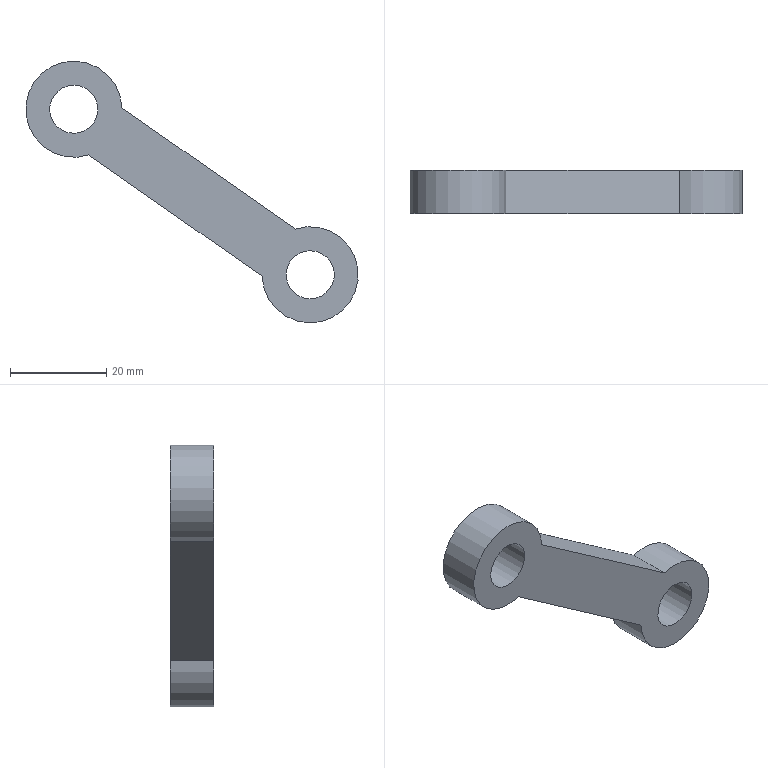Component | NX | CONNECTING_ROD_2 | 1 solid | 8 faces | box 69.15 x 9 x 54.41 mm | volume 8699 mm3 | cylinder 4 | plane 4 | commonest cylinder face diameters 20 x2 10 x2
STEP:
#1=CARTESIAN_POINT('',(0.,0.,0.));
#2=DIRECTION('',(0.,0.,1.));
#3=DIRECTION('',(1.,0.,0.));
#4=AXIS2_PLACEMENT_3D('',#1,#2,#3);
#5=CARTESIAN_POINT('',(-83.981,-59.005,124.741));
#6=VERTEX_POINT('',#5);
#7=CARTESIAN_POINT('',(-90.864,-59.005,114.911));
#8=VERTEX_POINT('',#7);
#9=CARTESIAN_POINT('',(-93.976,-59.005,124.415));
#10=DIRECTION('',(0.,-1.,0.));
#11=DIRECTION('',(0.8192,0.,-0.5736));
#12=AXIS2_PLACEMENT_3D('',#9,#10,#11);
#13=CIRCLE('',#12,10.);
#14=CARTESIAN_POINT('',(-93.976,-68.005,124.415));
#15=DIRECTION('',(0.,1.,0.));
#16=DIRECTION('',(-0.8192,0.,0.5736));
#17=AXIS2_PLACEMENT_3D('',#14,#15,#16);
#18=CYLINDRICAL_SURFACE('',#17,10.);
#19=CARTESIAN_POINT('',(3.142,9.));
#20=DIRECTION('',(-1.,0.));
#21=VECTOR('',#20,1.);
#22=LINE('',#19,#21);
#23=(GEOMETRIC_REPRESENTATION_CONTEXT(2)PARAMETRIC_REPRESENTATION_CONTEXT()REPRESENTATION_CONTEXT('',''));
#24=DEFINITIONAL_REPRESENTATION('',(#22),#23);
#25=PCURVE('',#18,#24);
#26=CARTESIAN_POINT('',(-93.976,-59.005,124.415));
#27=DIRECTION('',(0.,-1.,0.));
#28=DIRECTION('',(0.8192,0.,-0.5736));
#29=AXIS2_PLACEMENT_3D('',#26,#27,#28);
#30=PLANE('',#29);
#31=CARTESIAN_POINT('',(0.,0.));
#32=DIRECTION('',(1.,0.));
#33=AXIS2_PLACEMENT_2D('',#31,#32);
#34=CIRCLE('',#33,10.);
#35=(GEOMETRIC_REPRESENTATION_CONTEXT(2)PARAMETRIC_REPRESENTATION_CONTEXT()REPRESENTATION_CONTEXT('',''));
#36=DEFINITIONAL_REPRESENTATION('',(#34),#35);
#37=PCURVE('',#30,#36);
#38=SURFACE_CURVE('',#13,(#25,#37),.PCURVE_S1.);
#39=EDGE_CURVE('',#6,#8,#38,.T.);
#40=ORIENTED_EDGE('',*,*,#39,.T.);
#41=CARTESIAN_POINT('',(-90.864,-68.005,114.911));
#42=VERTEX_POINT('',#41);
#43=CARTESIAN_POINT('',(-90.864,-68.005,114.911));
#44=DIRECTION('',(0.,1.,0.));
#45=VECTOR('',#44,1.);
#46=LINE('',#43,#45);
#47=CARTESIAN_POINT('',(-2.498,0.));
#48=DIRECTION('',(0.,1.));
#49=VECTOR('',#48,1.);
#50=LINE('',#47,#49);
#51=(GEOMETRIC_REPRESENTATION_CONTEXT(2)PARAMETRIC_REPRESENTATION_CONTEXT()REPRESENTATION_CONTEXT('',''));
#52=DEFINITIONAL_REPRESENTATION('',(#50),#51);
#53=PCURVE('',#18,#52);
#54=CARTESIAN_POINT('',(-90.864,-68.005,114.911));
#55=DIRECTION('',(0.5736,0.,0.8192));
#56=DIRECTION('',(-0.8192,0.,0.5736));
#57=AXIS2_PLACEMENT_3D('',#54,#55,#56);
#58=PLANE('',#57);
#59=CARTESIAN_POINT('',(-0.,0.));
#60=DIRECTION('',(0.,-1.));
#61=VECTOR('',#60,1.);
#62=LINE('',#59,#61);
#63=(GEOMETRIC_REPRESENTATION_CONTEXT(2)PARAMETRIC_REPRESENTATION_CONTEXT()REPRESENTATION_CONTEXT('',''));
#64=DEFINITIONAL_REPRESENTATION('',(#62),#63);
#65=PCURVE('',#58,#64);
#66=SURFACE_CURVE('',#46,(#53,#65),.PCURVE_S1.);
#67=EDGE_CURVE('',#42,#8,#66,.T.);
#68=ORIENTED_EDGE('',*,*,#67,.F.);
#69=CARTESIAN_POINT('',(-83.981,-68.005,124.741));
#70=VERTEX_POINT('',#69);
#71=CARTESIAN_POINT('',(-93.976,-68.005,124.415));
#72=DIRECTION('',(0.,-1.,0.));
#73=DIRECTION('',(0.8192,0.,-0.5736));
#74=AXIS2_PLACEMENT_3D('',#71,#72,#73);
#75=CIRCLE('',#74,10.);
#76=CARTESIAN_POINT('',(3.142,0.));
#77=DIRECTION('',(-1.,0.));
#78=VECTOR('',#77,1.);
#79=LINE('',#76,#78);
#80=(GEOMETRIC_REPRESENTATION_CONTEXT(2)PARAMETRIC_REPRESENTATION_CONTEXT()REPRESENTATION_CONTEXT('',''));
#81=DEFINITIONAL_REPRESENTATION('',(#79),#80);
#82=PCURVE('',#18,#81);
#83=CARTESIAN_POINT('',(-93.976,-68.005,124.415));
#84=DIRECTION('',(0.,-1.,0.));
#85=DIRECTION('',(0.8192,0.,-0.5736));
#86=AXIS2_PLACEMENT_3D('',#83,#84,#85);
#87=PLANE('',#86);
#88=CARTESIAN_POINT('',(0.,0.));
#89=DIRECTION('',(1.,0.));
#90=AXIS2_PLACEMENT_2D('',#88,#89);
#91=CIRCLE('',#90,10.);
#92=(GEOMETRIC_REPRESENTATION_CONTEXT(2)PARAMETRIC_REPRESENTATION_CONTEXT()REPRESENTATION_CONTEXT('',''));
#93=DEFINITIONAL_REPRESENTATION('',(#91),#92);
#94=PCURVE('',#87,#93);
#95=SURFACE_CURVE('',#75,(#82,#94),.PCURVE_S1.);
#96=EDGE_CURVE('',#70,#42,#95,.T.);
#97=ORIENTED_EDGE('',*,*,#96,.F.);
#98=CARTESIAN_POINT('',(-83.981,-68.005,124.741));
#99=DIRECTION('',(0.,1.,0.));
#100=VECTOR('',#99,1.);
#101=LINE('',#98,#100);
#102=CARTESIAN_POINT('',(2.498,0.));
#103=DIRECTION('',(0.,1.));
#104=VECTOR('',#103,1.);
#105=LINE('',#102,#104);
#106=(GEOMETRIC_REPRESENTATION_CONTEXT(2)PARAMETRIC_REPRESENTATION_CONTEXT()REPRESENTATION_CONTEXT('',''));
#107=DEFINITIONAL_REPRESENTATION('',(#105),#106);
#108=PCURVE('',#18,#107);
#109=CARTESIAN_POINT('',(-47.938,-68.005,99.504));
#110=DIRECTION('',(-0.5736,0.,-0.8192));
#111=DIRECTION('',(0.8192,0.,-0.5736));
#112=AXIS2_PLACEMENT_3D('',#109,#110,#111);
#113=PLANE('',#112);
#114=CARTESIAN_POINT('',(-44.,0.));
#115=DIRECTION('',(0.,-1.));
#116=VECTOR('',#115,1.);
#117=LINE('',#114,#116);
#118=(GEOMETRIC_REPRESENTATION_CONTEXT(2)PARAMETRIC_REPRESENTATION_CONTEXT()REPRESENTATION_CONTEXT('',''));
#119=DEFINITIONAL_REPRESENTATION('',(#117),#118);
#120=PCURVE('',#113,#119);
#121=SURFACE_CURVE('',#101,(#108,#120),.PCURVE_S1.);
#122=EDGE_CURVE('',#70,#6,#121,.T.);
#123=ORIENTED_EDGE('',*,*,#122,.T.);
#124=EDGE_LOOP('',(#40,#68,#97,#123));
#125=FACE_BOUND('',#124,.T.);
#126=ADVANCED_FACE('',(#125),#18,.T.);
#127=CARTESIAN_POINT('',(-54.821,-59.005,89.674));
#128=VERTEX_POINT('',#127);
#129=CARTESIAN_POINT('',(-90.864,-59.005,114.911));
#130=DIRECTION('',(0.8192,0.,-0.5736));
#131=VECTOR('',#130,1.);
#132=LINE('',#129,#131);
#133=CARTESIAN_POINT('',(0.,-9.));
#134=DIRECTION('',(-1.,0.));
#135=VECTOR('',#134,1.);
#136=LINE('',#133,#135);
#137=(GEOMETRIC_REPRESENTATION_CONTEXT(2)PARAMETRIC_REPRESENTATION_CONTEXT()REPRESENTATION_CONTEXT('',''));
#138=DEFINITIONAL_REPRESENTATION('',(#136),#137);
#139=PCURVE('',#58,#138);
#140=CARTESIAN_POINT('',(8.,-6.));
#141=DIRECTION('',(1.,0.));
#142=VECTOR('',#141,1.);
#143=LINE('',#140,#142);
#144=(GEOMETRIC_REPRESENTATION_CONTEXT(2)PARAMETRIC_REPRESENTATION_CONTEXT()REPRESENTATION_CONTEXT('',''));
#145=DEFINITIONAL_REPRESENTATION('',(#143),#144);
#146=PCURVE('',#30,#145);
#147=SURFACE_CURVE('',#132,(#139,#146),.PCURVE_S1.);
#148=EDGE_CURVE('',#8,#128,#147,.T.);
#149=ORIENTED_EDGE('',*,*,#148,.T.);
#150=CARTESIAN_POINT('',(-54.821,-68.005,89.674));
#151=VERTEX_POINT('',#150);
#152=CARTESIAN_POINT('',(-54.821,-68.005,89.674));
#153=DIRECTION('',(0.,1.,0.));
#154=VECTOR('',#153,1.);
#155=LINE('',#152,#154);
#156=CARTESIAN_POINT('',(-44.,0.));
#157=DIRECTION('',(0.,-1.));
#158=VECTOR('',#157,1.);
#159=LINE('',#156,#158);
#160=(GEOMETRIC_REPRESENTATION_CONTEXT(2)PARAMETRIC_REPRESENTATION_CONTEXT()REPRESENTATION_CONTEXT('',''));
#161=DEFINITIONAL_REPRESENTATION('',(#159),#160);
#162=PCURVE('',#58,#161);
#163=CARTESIAN_POINT('',(-44.827,-68.005,90.));
#164=DIRECTION('',(0.,1.,0.));
#165=DIRECTION('',(-0.8192,0.,0.5736));
#166=AXIS2_PLACEMENT_3D('',#163,#164,#165);
#167=CYLINDRICAL_SURFACE('',#166,10.);
#168=CARTESIAN_POINT('',(5.64,0.));
#169=DIRECTION('',(0.,1.));
#170=VECTOR('',#169,1.);
#171=LINE('',#168,#170);
#172=(GEOMETRIC_REPRESENTATION_CONTEXT(2)PARAMETRIC_REPRESENTATION_CONTEXT()REPRESENTATION_CONTEXT('',''));
#173=DEFINITIONAL_REPRESENTATION('',(#171),#172);
#174=PCURVE('',#167,#173);
#175=SURFACE_CURVE('',#155,(#162,#174),.PCURVE_S1.);
#176=EDGE_CURVE('',#151,#128,#175,.T.);
#177=ORIENTED_EDGE('',*,*,#176,.F.);
#178=CARTESIAN_POINT('',(-90.864,-68.005,114.911));
#179=DIRECTION('',(0.8192,0.,-0.5736));
#180=VECTOR('',#179,1.);
#181=LINE('',#178,#180);
#182=CARTESIAN_POINT('',(0.,0.));
#183=DIRECTION('',(-1.,0.));
#184=VECTOR('',#183,1.);
#185=LINE('',#182,#184);
#186=(GEOMETRIC_REPRESENTATION_CONTEXT(2)PARAMETRIC_REPRESENTATION_CONTEXT()REPRESENTATION_CONTEXT('',''));
#187=DEFINITIONAL_REPRESENTATION('',(#185),#186);
#188=PCURVE('',#58,#187);
#189=CARTESIAN_POINT('',(8.,-6.));
#190=DIRECTION('',(1.,0.));
#191=VECTOR('',#190,1.);
#192=LINE('',#189,#191);
#193=(GEOMETRIC_REPRESENTATION_CONTEXT(2)PARAMETRIC_REPRESENTATION_CONTEXT()REPRESENTATION_CONTEXT('',''));
#194=DEFINITIONAL_REPRESENTATION('',(#192),#193);
#195=PCURVE('',#87,#194);
#196=SURFACE_CURVE('',#181,(#188,#195),.PCURVE_S1.);
#197=EDGE_CURVE('',#42,#151,#196,.T.);
#198=ORIENTED_EDGE('',*,*,#197,.F.);
#199=ORIENTED_EDGE('',*,*,#67,.T.);
#200=EDGE_LOOP('',(#149,#177,#198,#199));
#201=FACE_BOUND('',#200,.T.);
#202=ADVANCED_FACE('',(#201),#58,.F.);
#203=CARTESIAN_POINT('',(-47.938,-59.005,99.504));
#204=VERTEX_POINT('',#203);
#205=CARTESIAN_POINT('',(-44.827,-59.005,90.));
#206=DIRECTION('',(0.,-1.,0.));
#207=DIRECTION('',(0.8192,0.,-0.5736));
#208=AXIS2_PLACEMENT_3D('',#205,#206,#207);
#209=CIRCLE('',#208,10.);
#210=CARTESIAN_POINT('',(9.425,9.));
#211=DIRECTION('',(-1.,0.));
#212=VECTOR('',#211,1.);
#213=LINE('',#210,#212);
#214=(GEOMETRIC_REPRESENTATION_CONTEXT(2)PARAMETRIC_REPRESENTATION_CONTEXT()REPRESENTATION_CONTEXT('',''));
#215=DEFINITIONAL_REPRESENTATION('',(#213),#214);
#216=PCURVE('',#167,#215);
#217=CARTESIAN_POINT('',(60.,-0.));
#218=DIRECTION('',(1.,0.));
#219=AXIS2_PLACEMENT_2D('',#217,#218);
#220=CIRCLE('',#219,10.);
#221=(GEOMETRIC_REPRESENTATION_CONTEXT(2)PARAMETRIC_REPRESENTATION_CONTEXT()REPRESENTATION_CONTEXT('',''));
#222=DEFINITIONAL_REPRESENTATION('',(#220),#221);
#223=PCURVE('',#30,#222);
#224=SURFACE_CURVE('',#209,(#216,#223),.PCURVE_S1.);
#225=EDGE_CURVE('',#128,#204,#224,.T.);
#226=ORIENTED_EDGE('',*,*,#225,.T.);
#227=CARTESIAN_POINT('',(-47.938,-68.005,99.504));
#228=VERTEX_POINT('',#227);
#229=CARTESIAN_POINT('',(-47.938,-68.005,99.504));
#230=DIRECTION('',(0.,1.,0.));
#231=VECTOR('',#230,1.);
#232=LINE('',#229,#231);
#233=CARTESIAN_POINT('',(0.6435,0.));
#234=DIRECTION('',(0.,1.));
#235=VECTOR('',#234,1.);
#236=LINE('',#233,#235);
#237=(GEOMETRIC_REPRESENTATION_CONTEXT(2)PARAMETRIC_REPRESENTATION_CONTEXT()REPRESENTATION_CONTEXT('',''));
#238=DEFINITIONAL_REPRESENTATION('',(#236),#237);
#239=PCURVE('',#167,#238);
#240=CARTESIAN_POINT('',(0.,0.));
#241=DIRECTION('',(0.,-1.));
#242=VECTOR('',#241,1.);
#243=LINE('',#240,#242);
#244=(GEOMETRIC_REPRESENTATION_CONTEXT(2)PARAMETRIC_REPRESENTATION_CONTEXT()REPRESENTATION_CONTEXT('',''));
#245=DEFINITIONAL_REPRESENTATION('',(#243),#244);
#246=PCURVE('',#113,#245);
#247=SURFACE_CURVE('',#232,(#239,#246),.PCURVE_S1.);
#248=EDGE_CURVE('',#228,#204,#247,.T.);
#249=ORIENTED_EDGE('',*,*,#248,.F.);
#250=CARTESIAN_POINT('',(-44.827,-68.005,90.));
#251=DIRECTION('',(0.,-1.,0.));
#252=DIRECTION('',(0.8192,0.,-0.5736));
#253=AXIS2_PLACEMENT_3D('',#250,#251,#252);
#254=CIRCLE('',#253,10.);
#255=CARTESIAN_POINT('',(9.425,0.));
#256=DIRECTION('',(-1.,0.));
#257=VECTOR('',#256,1.);
#258=LINE('',#255,#257);
#259=(GEOMETRIC_REPRESENTATION_CONTEXT(2)PARAMETRIC_REPRESENTATION_CONTEXT()REPRESENTATION_CONTEXT('',''));
#260=DEFINITIONAL_REPRESENTATION('',(#258),#259);
#261=PCURVE('',#167,#260);
#262=CARTESIAN_POINT('',(60.,-0.));
#263=DIRECTION('',(1.,0.));
#264=AXIS2_PLACEMENT_2D('',#262,#263);
#265=CIRCLE('',#264,10.);
#266=(GEOMETRIC_REPRESENTATION_CONTEXT(2)PARAMETRIC_REPRESENTATION_CONTEXT()REPRESENTATION_CONTEXT('',''));
#267=DEFINITIONAL_REPRESENTATION('',(#265),#266);
#268=PCURVE('',#87,#267);
#269=SURFACE_CURVE('',#254,(#261,#268),.PCURVE_S1.);
#270=EDGE_CURVE('',#151,#228,#269,.T.);
#271=ORIENTED_EDGE('',*,*,#270,.F.);
#272=ORIENTED_EDGE('',*,*,#176,.T.);
#273=EDGE_LOOP('',(#226,#249,#271,#272));
#274=FACE_BOUND('',#273,.T.);
#275=ADVANCED_FACE('',(#274),#167,.T.);
#276=CARTESIAN_POINT('',(-89.88,-68.005,121.547));
#277=VERTEX_POINT('',#276);
#278=CARTESIAN_POINT('',(-93.976,-68.005,124.415));
#279=DIRECTION('',(0.,-1.,0.));
#280=DIRECTION('',(0.8192,0.,-0.5736));
#281=AXIS2_PLACEMENT_3D('',#278,#279,#280);
#282=CIRCLE('',#281,5.);
#283=CARTESIAN_POINT('',(-93.976,-68.005,124.415));
#284=DIRECTION('',(0.,1.,0.));
#285=DIRECTION('',(-0.8192,0.,0.5736));
#286=AXIS2_PLACEMENT_3D('',#283,#284,#285);
#287=CYLINDRICAL_SURFACE('',#286,5.);
#288=CARTESIAN_POINT('',(9.425,0.));
#289=DIRECTION('',(-1.,0.));
#290=VECTOR('',#289,1.);
#291=LINE('',#288,#290);
#292=(GEOMETRIC_REPRESENTATION_CONTEXT(2)PARAMETRIC_REPRESENTATION_CONTEXT()REPRESENTATION_CONTEXT('',''));
#293=DEFINITIONAL_REPRESENTATION('',(#291),#292);
#294=PCURVE('',#287,#293);
#295=CARTESIAN_POINT('',(0.,0.));
#296=DIRECTION('',(1.,0.));
#297=AXIS2_PLACEMENT_2D('',#295,#296);
#298=CIRCLE('',#297,5.);
#299=(GEOMETRIC_REPRESENTATION_CONTEXT(2)PARAMETRIC_REPRESENTATION_CONTEXT()REPRESENTATION_CONTEXT('',''));
#300=DEFINITIONAL_REPRESENTATION('',(#298),#299);
#301=PCURVE('',#87,#300);
#302=SURFACE_CURVE('',#282,(#294,#301),.PCURVE_S1.);
#303=EDGE_CURVE('',#277,#277,#302,.T.);
#304=ORIENTED_EDGE('',*,*,#303,.F.);
#305=CARTESIAN_POINT('',(-89.88,-59.005,121.547));
#306=VERTEX_POINT('',#305);
#307=CARTESIAN_POINT('',(-89.88,-68.005,121.547));
#308=CARTESIAN_POINT('',(-89.88,-59.005,121.547));
#309=B_SPLINE_CURVE_WITH_KNOTS('',1,(#307,#308),.UNSPECIFIED.,.F.,.F.,(2,2),(0.,9.),.PIECEWISE_BEZIER_KNOTS.);
#310=CARTESIAN_POINT('',(9.425,0.));
#311=DIRECTION('',(0.,1.));
#312=VECTOR('',#311,1.);
#313=LINE('',#310,#312);
#314=(GEOMETRIC_REPRESENTATION_CONTEXT(2)PARAMETRIC_REPRESENTATION_CONTEXT()REPRESENTATION_CONTEXT('',''));
#315=DEFINITIONAL_REPRESENTATION('',(#313),#314);
#316=PCURVE('',#287,#315);
#317=CARTESIAN_POINT('',(3.142,0.));
#318=DIRECTION('',(0.,1.));
#319=VECTOR('',#318,1.);
#320=LINE('',#317,#319);
#321=(GEOMETRIC_REPRESENTATION_CONTEXT(2)PARAMETRIC_REPRESENTATION_CONTEXT()REPRESENTATION_CONTEXT('',''));
#322=DEFINITIONAL_REPRESENTATION('',(#320),#321);
#323=PCURVE('',#287,#322);
#324=SEAM_CURVE('',#309,(#316,#323),.PCURVE_S1.);
#325=EDGE_CURVE('',#277,#306,#324,.T.);
#326=ORIENTED_EDGE('',*,*,#325,.T.);
#327=CARTESIAN_POINT('',(-93.976,-59.005,124.415));
#328=DIRECTION('',(0.,-1.,0.));
#329=DIRECTION('',(0.8192,0.,-0.5736));
#330=AXIS2_PLACEMENT_3D('',#327,#328,#329);
#331=CIRCLE('',#330,5.);
#332=CARTESIAN_POINT('',(9.425,9.));
#333=DIRECTION('',(-1.,0.));
#334=VECTOR('',#333,1.);
#335=LINE('',#332,#334);
#336=(GEOMETRIC_REPRESENTATION_CONTEXT(2)PARAMETRIC_REPRESENTATION_CONTEXT()REPRESENTATION_CONTEXT('',''));
#337=DEFINITIONAL_REPRESENTATION('',(#335),#336);
#338=PCURVE('',#287,#337);
#339=CARTESIAN_POINT('',(0.,0.));
#340=DIRECTION('',(1.,0.));
#341=AXIS2_PLACEMENT_2D('',#339,#340);
#342=CIRCLE('',#341,5.);
#343=(GEOMETRIC_REPRESENTATION_CONTEXT(2)PARAMETRIC_REPRESENTATION_CONTEXT()REPRESENTATION_CONTEXT('',''));
#344=DEFINITIONAL_REPRESENTATION('',(#342),#343);
#345=PCURVE('',#30,#344);
#346=SURFACE_CURVE('',#331,(#338,#345),.PCURVE_S1.);
#347=EDGE_CURVE('',#306,#306,#346,.T.);
#348=ORIENTED_EDGE('',*,*,#347,.T.);
#349=ORIENTED_EDGE('',*,*,#325,.F.);
#350=EDGE_LOOP('',(#304,#326,#348,#349));
#351=FACE_BOUND('',#350,.F.);
#352=ADVANCED_FACE('',(#351),#287,.F.);
#353=CARTESIAN_POINT('',(-47.938,-59.005,99.504));
#354=DIRECTION('',(-0.8192,0.,0.5736));
#355=VECTOR('',#354,1.);
#356=LINE('',#353,#355);
#357=CARTESIAN_POINT('',(0.,-9.));
#358=DIRECTION('',(-1.,0.));
#359=VECTOR('',#358,1.);
#360=LINE('',#357,#359);
#361=(GEOMETRIC_REPRESENTATION_CONTEXT(2)PARAMETRIC_REPRESENTATION_CONTEXT()REPRESENTATION_CONTEXT('',''));
#362=DEFINITIONAL_REPRESENTATION('',(#360),#361);
#363=PCURVE('',#113,#362);
#364=CARTESIAN_POINT('',(52.,6.));
#365=DIRECTION('',(-1.,0.));
#366=VECTOR('',#365,1.);
#367=LINE('',#364,#366);
#368=(GEOMETRIC_REPRESENTATION_CONTEXT(2)PARAMETRIC_REPRESENTATION_CONTEXT()REPRESENTATION_CONTEXT('',''));
#369=DEFINITIONAL_REPRESENTATION('',(#367),#368);
#370=PCURVE('',#30,#369);
#371=SURFACE_CURVE('',#356,(#363,#370),.PCURVE_S1.);
#372=EDGE_CURVE('',#204,#6,#371,.T.);
#373=ORIENTED_EDGE('',*,*,#372,.T.);
#374=ORIENTED_EDGE('',*,*,#122,.F.);
#375=CARTESIAN_POINT('',(-47.938,-68.005,99.504));
#376=DIRECTION('',(-0.8192,0.,0.5736));
#377=VECTOR('',#376,1.);
#378=LINE('',#375,#377);
#379=CARTESIAN_POINT('',(0.,0.));
#380=DIRECTION('',(-1.,0.));
#381=VECTOR('',#380,1.);
#382=LINE('',#379,#381);
#383=(GEOMETRIC_REPRESENTATION_CONTEXT(2)PARAMETRIC_REPRESENTATION_CONTEXT()REPRESENTATION_CONTEXT('',''));
#384=DEFINITIONAL_REPRESENTATION('',(#382),#383);
#385=PCURVE('',#113,#384);
#386=CARTESIAN_POINT('',(52.,6.));
#387=DIRECTION('',(-1.,0.));
#388=VECTOR('',#387,1.);
#389=LINE('',#386,#388);
#390=(GEOMETRIC_REPRESENTATION_CONTEXT(2)PARAMETRIC_REPRESENTATION_CONTEXT()REPRESENTATION_CONTEXT('',''));
#391=DEFINITIONAL_REPRESENTATION('',(#389),#390);
#392=PCURVE('',#87,#391);
#393=SURFACE_CURVE('',#378,(#385,#392),.PCURVE_S1.);
#394=EDGE_CURVE('',#228,#70,#393,.T.);
#395=ORIENTED_EDGE('',*,*,#394,.F.);
#396=ORIENTED_EDGE('',*,*,#248,.T.);
#397=EDGE_LOOP('',(#373,#374,#395,#396));
#398=FACE_BOUND('',#397,.T.);
#399=ADVANCED_FACE('',(#398),#113,.F.);
#400=CARTESIAN_POINT('',(-40.731,-68.005,87.132));
#401=VERTEX_POINT('',#400);
#402=CARTESIAN_POINT('',(-44.827,-68.005,90.));
#403=DIRECTION('',(0.,-1.,0.));
#404=DIRECTION('',(0.8192,0.,-0.5736));
#405=AXIS2_PLACEMENT_3D('',#402,#403,#404);
#406=CIRCLE('',#405,5.);
#407=CARTESIAN_POINT('',(-44.827,-68.005,90.));
#408=DIRECTION('',(0.,1.,0.));
#409=DIRECTION('',(-0.8192,0.,0.5736));
#410=AXIS2_PLACEMENT_3D('',#407,#408,#409);
#411=CYLINDRICAL_SURFACE('',#410,5.);
#412=CARTESIAN_POINT('',(9.425,0.));
#413=DIRECTION('',(-1.,0.));
#414=VECTOR('',#413,1.);
#415=LINE('',#412,#414);
#416=(GEOMETRIC_REPRESENTATION_CONTEXT(2)PARAMETRIC_REPRESENTATION_CONTEXT()REPRESENTATION_CONTEXT('',''));
#417=DEFINITIONAL_REPRESENTATION('',(#415),#416);
#418=PCURVE('',#411,#417);
#419=CARTESIAN_POINT('',(60.,-0.));
#420=DIRECTION('',(1.,0.));
#421=AXIS2_PLACEMENT_2D('',#419,#420);
#422=CIRCLE('',#421,5.);
#423=(GEOMETRIC_REPRESENTATION_CONTEXT(2)PARAMETRIC_REPRESENTATION_CONTEXT()REPRESENTATION_CONTEXT('',''));
#424=DEFINITIONAL_REPRESENTATION('',(#422),#423);
#425=PCURVE('',#87,#424);
#426=SURFACE_CURVE('',#406,(#418,#425),.PCURVE_S1.);
#427=EDGE_CURVE('',#401,#401,#426,.T.);
#428=ORIENTED_EDGE('',*,*,#427,.F.);
#429=CARTESIAN_POINT('',(-40.731,-59.005,87.132));
#430=VERTEX_POINT('',#429);
#431=CARTESIAN_POINT('',(-40.731,-68.005,87.132));
#432=CARTESIAN_POINT('',(-40.731,-59.005,87.132));
#433=B_SPLINE_CURVE_WITH_KNOTS('',1,(#431,#432),.UNSPECIFIED.,.F.,.F.,(2,2),(0.,9.),.PIECEWISE_BEZIER_KNOTS.);
#434=CARTESIAN_POINT('',(9.425,0.));
#435=DIRECTION('',(0.,1.));
#436=VECTOR('',#435,1.);
#437=LINE('',#434,#436);
#438=(GEOMETRIC_REPRESENTATION_CONTEXT(2)PARAMETRIC_REPRESENTATION_CONTEXT()REPRESENTATION_CONTEXT('',''));
#439=DEFINITIONAL_REPRESENTATION('',(#437),#438);
#440=PCURVE('',#411,#439);
#441=CARTESIAN_POINT('',(3.142,0.));
#442=DIRECTION('',(0.,1.));
#443=VECTOR('',#442,1.);
#444=LINE('',#441,#443);
#445=(GEOMETRIC_REPRESENTATION_CONTEXT(2)PARAMETRIC_REPRESENTATION_CONTEXT()REPRESENTATION_CONTEXT('',''));
#446=DEFINITIONAL_REPRESENTATION('',(#444),#445);
#447=PCURVE('',#411,#446);
#448=SEAM_CURVE('',#433,(#440,#447),.PCURVE_S1.);
#449=EDGE_CURVE('',#401,#430,#448,.T.);
#450=ORIENTED_EDGE('',*,*,#449,.T.);
#451=CARTESIAN_POINT('',(-44.827,-59.005,90.));
#452=DIRECTION('',(0.,-1.,0.));
#453=DIRECTION('',(0.8192,0.,-0.5736));
#454=AXIS2_PLACEMENT_3D('',#451,#452,#453);
#455=CIRCLE('',#454,5.);
#456=CARTESIAN_POINT('',(9.425,9.));
#457=DIRECTION('',(-1.,0.));
#458=VECTOR('',#457,1.);
#459=LINE('',#456,#458);
#460=(GEOMETRIC_REPRESENTATION_CONTEXT(2)PARAMETRIC_REPRESENTATION_CONTEXT()REPRESENTATION_CONTEXT('',''));
#461=DEFINITIONAL_REPRESENTATION('',(#459),#460);
#462=PCURVE('',#411,#461);
#463=CARTESIAN_POINT('',(60.,-0.));
#464=DIRECTION('',(1.,0.));
#465=AXIS2_PLACEMENT_2D('',#463,#464);
#466=CIRCLE('',#465,5.);
#467=(GEOMETRIC_REPRESENTATION_CONTEXT(2)PARAMETRIC_REPRESENTATION_CONTEXT()REPRESENTATION_CONTEXT('',''));
#468=DEFINITIONAL_REPRESENTATION('',(#466),#467);
#469=PCURVE('',#30,#468);
#470=SURFACE_CURVE('',#455,(#462,#469),.PCURVE_S1.);
#471=EDGE_CURVE('',#430,#430,#470,.T.);
#472=ORIENTED_EDGE('',*,*,#471,.T.);
#473=ORIENTED_EDGE('',*,*,#449,.F.);
#474=EDGE_LOOP('',(#428,#450,#472,#473));
#475=FACE_BOUND('',#474,.F.);
#476=ADVANCED_FACE('',(#475),#411,.F.);
#477=ORIENTED_EDGE('',*,*,#96,.T.);
#478=ORIENTED_EDGE('',*,*,#197,.T.);
#479=ORIENTED_EDGE('',*,*,#270,.T.);
#480=ORIENTED_EDGE('',*,*,#394,.T.);
#481=EDGE_LOOP('',(#477,#478,#479,#480));
#482=FACE_BOUND('',#481,.T.);
#483=ORIENTED_EDGE('',*,*,#303,.F.);
#484=EDGE_LOOP('',(#483));
#485=FACE_BOUND('',#484,.T.);
#486=ORIENTED_EDGE('',*,*,#427,.F.);
#487=EDGE_LOOP('',(#486));
#488=FACE_BOUND('',#487,.T.);
#489=ADVANCED_FACE('',(#482,#485,#488),#87,.T.);
#490=ORIENTED_EDGE('',*,*,#39,.F.);
#491=ORIENTED_EDGE('',*,*,#372,.F.);
#492=ORIENTED_EDGE('',*,*,#225,.F.);
#493=ORIENTED_EDGE('',*,*,#148,.F.);
#494=EDGE_LOOP('',(#490,#491,#492,#493));
#495=FACE_BOUND('',#494,.T.);
#496=ORIENTED_EDGE('',*,*,#347,.T.);
#497=EDGE_LOOP('',(#496));
#498=FACE_BOUND('',#497,.T.);
#499=ORIENTED_EDGE('',*,*,#471,.T.);
#500=EDGE_LOOP('',(#499));
#501=FACE_BOUND('',#500,.T.);
#502=ADVANCED_FACE('',(#495,#498,#501),#30,.F.);
#503=CLOSED_SHELL('',(#126,#202,#275,#352,#399,#476,#489,#502));
#504=MANIFOLD_SOLID_BREP('',#503);
#505=(LENGTH_UNIT()NAMED_UNIT(*)SI_UNIT(.MILLI.,.METRE.));
#506=UNCERTAINTY_MEASURE_WITH_UNIT(LENGTH_MEASURE(0.000002),#505,'','');
#507=(NAMED_UNIT(*)PLANE_ANGLE_UNIT()SI_UNIT($,.RADIAN.));
#508=(NAMED_UNIT(*)SI_UNIT($,.STERADIAN.)SOLID_ANGLE_UNIT());
#509=(GEOMETRIC_REPRESENTATION_CONTEXT(3)GLOBAL_UNCERTAINTY_ASSIGNED_CONTEXT((#506))GLOBAL_UNIT_ASSIGNED_CONTEXT((#505,#507,#508))REPRESENTATION_CONTEXT('',''));
#510=ADVANCED_BREP_SHAPE_REPRESENTATION('',(#4,#504),#509);